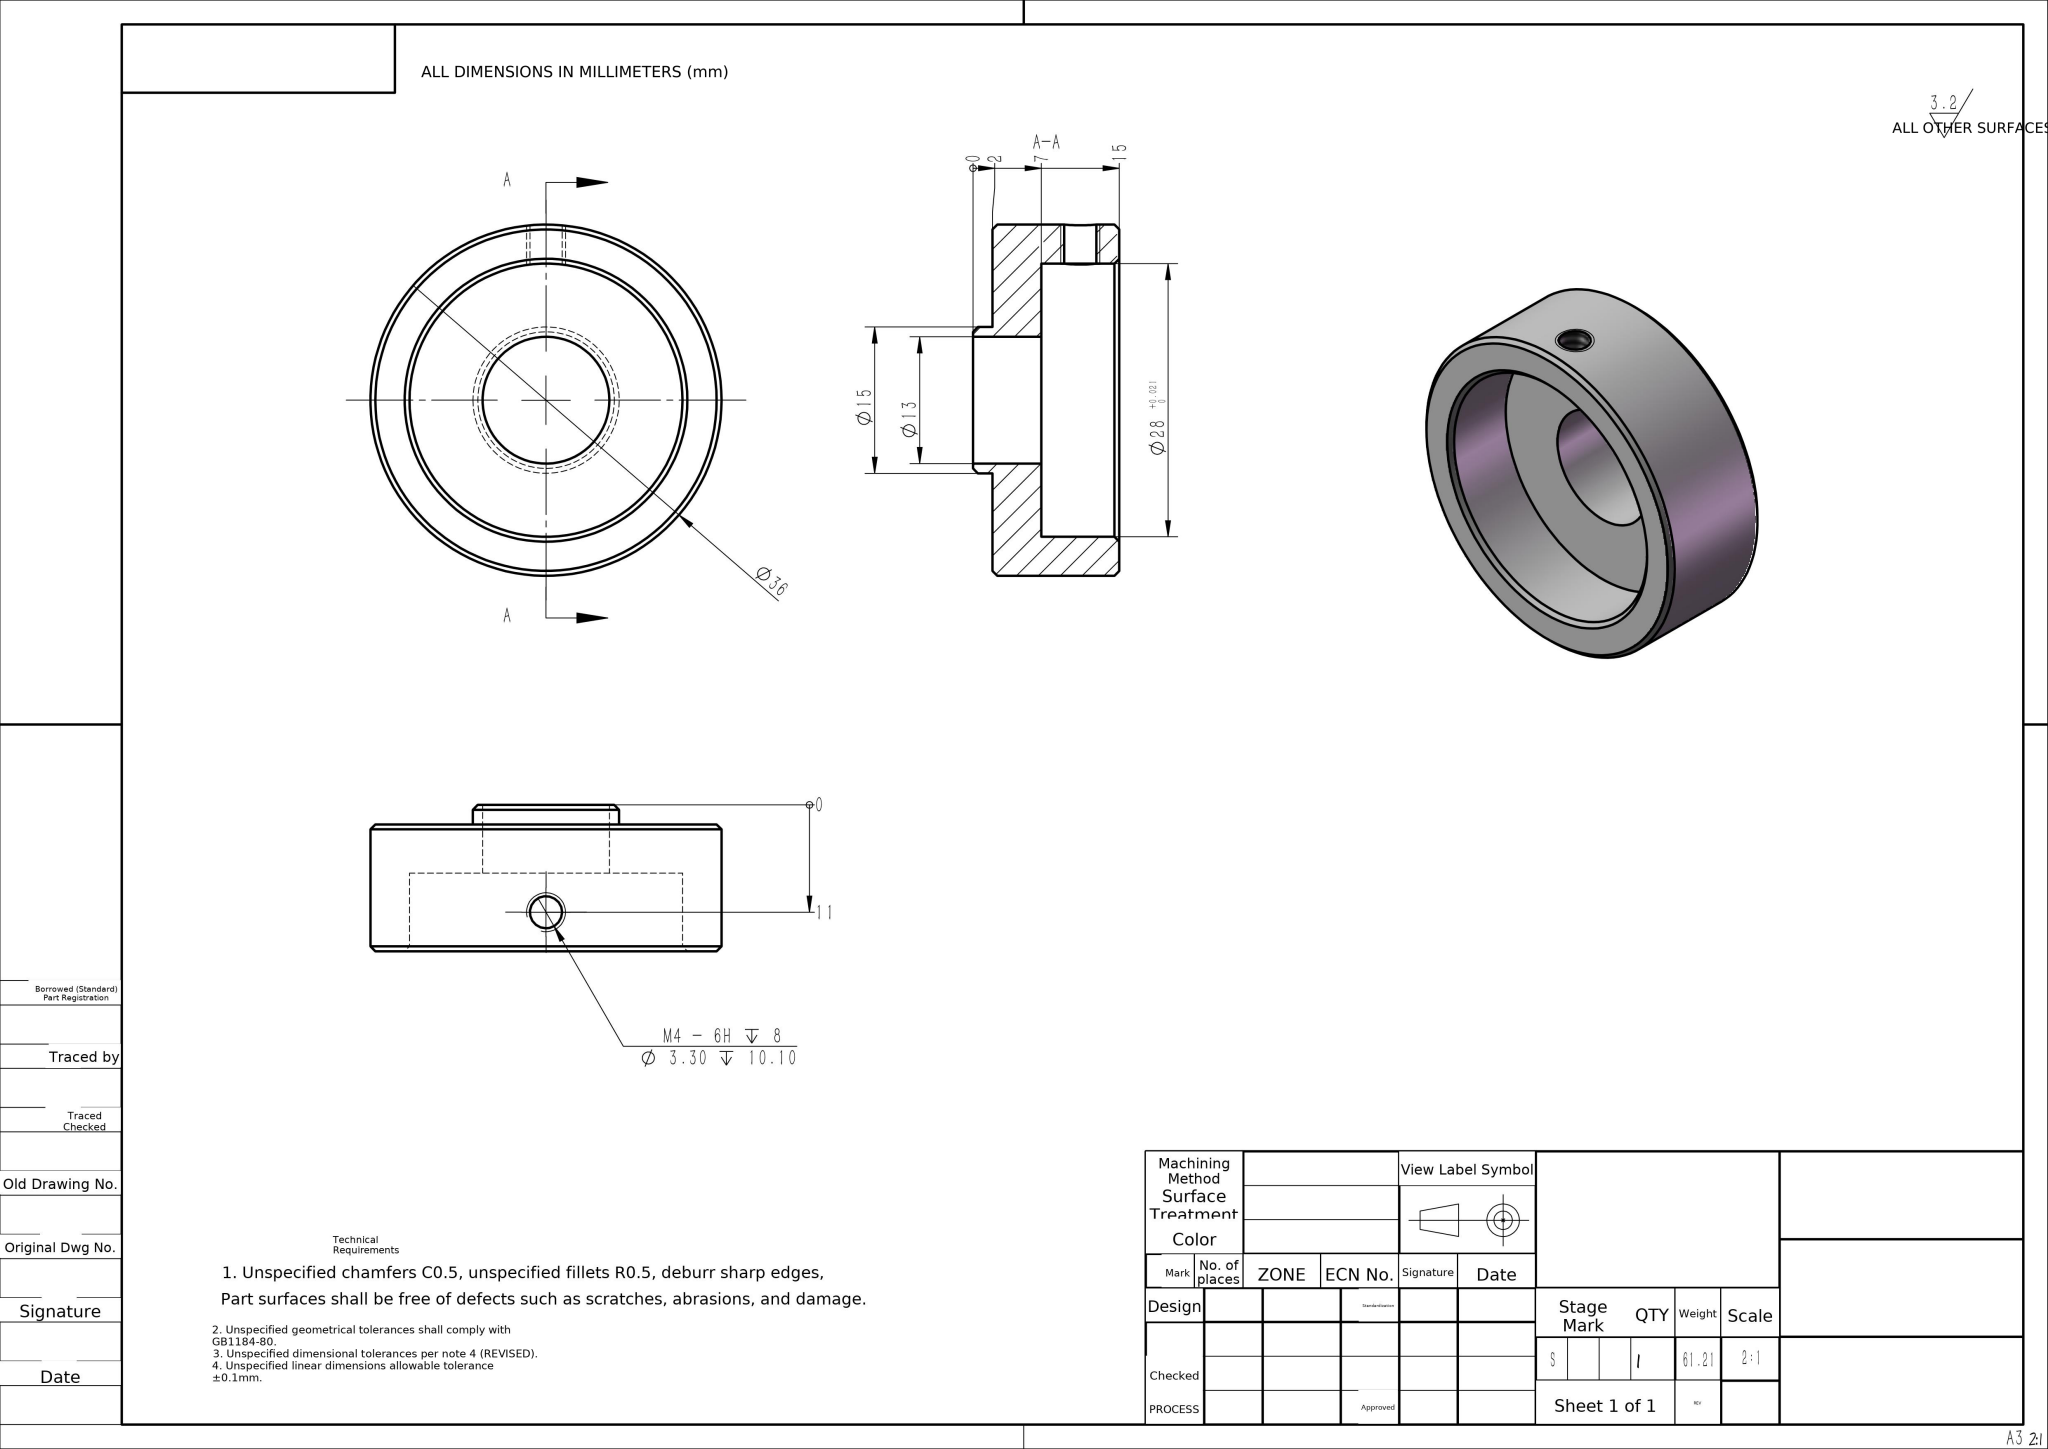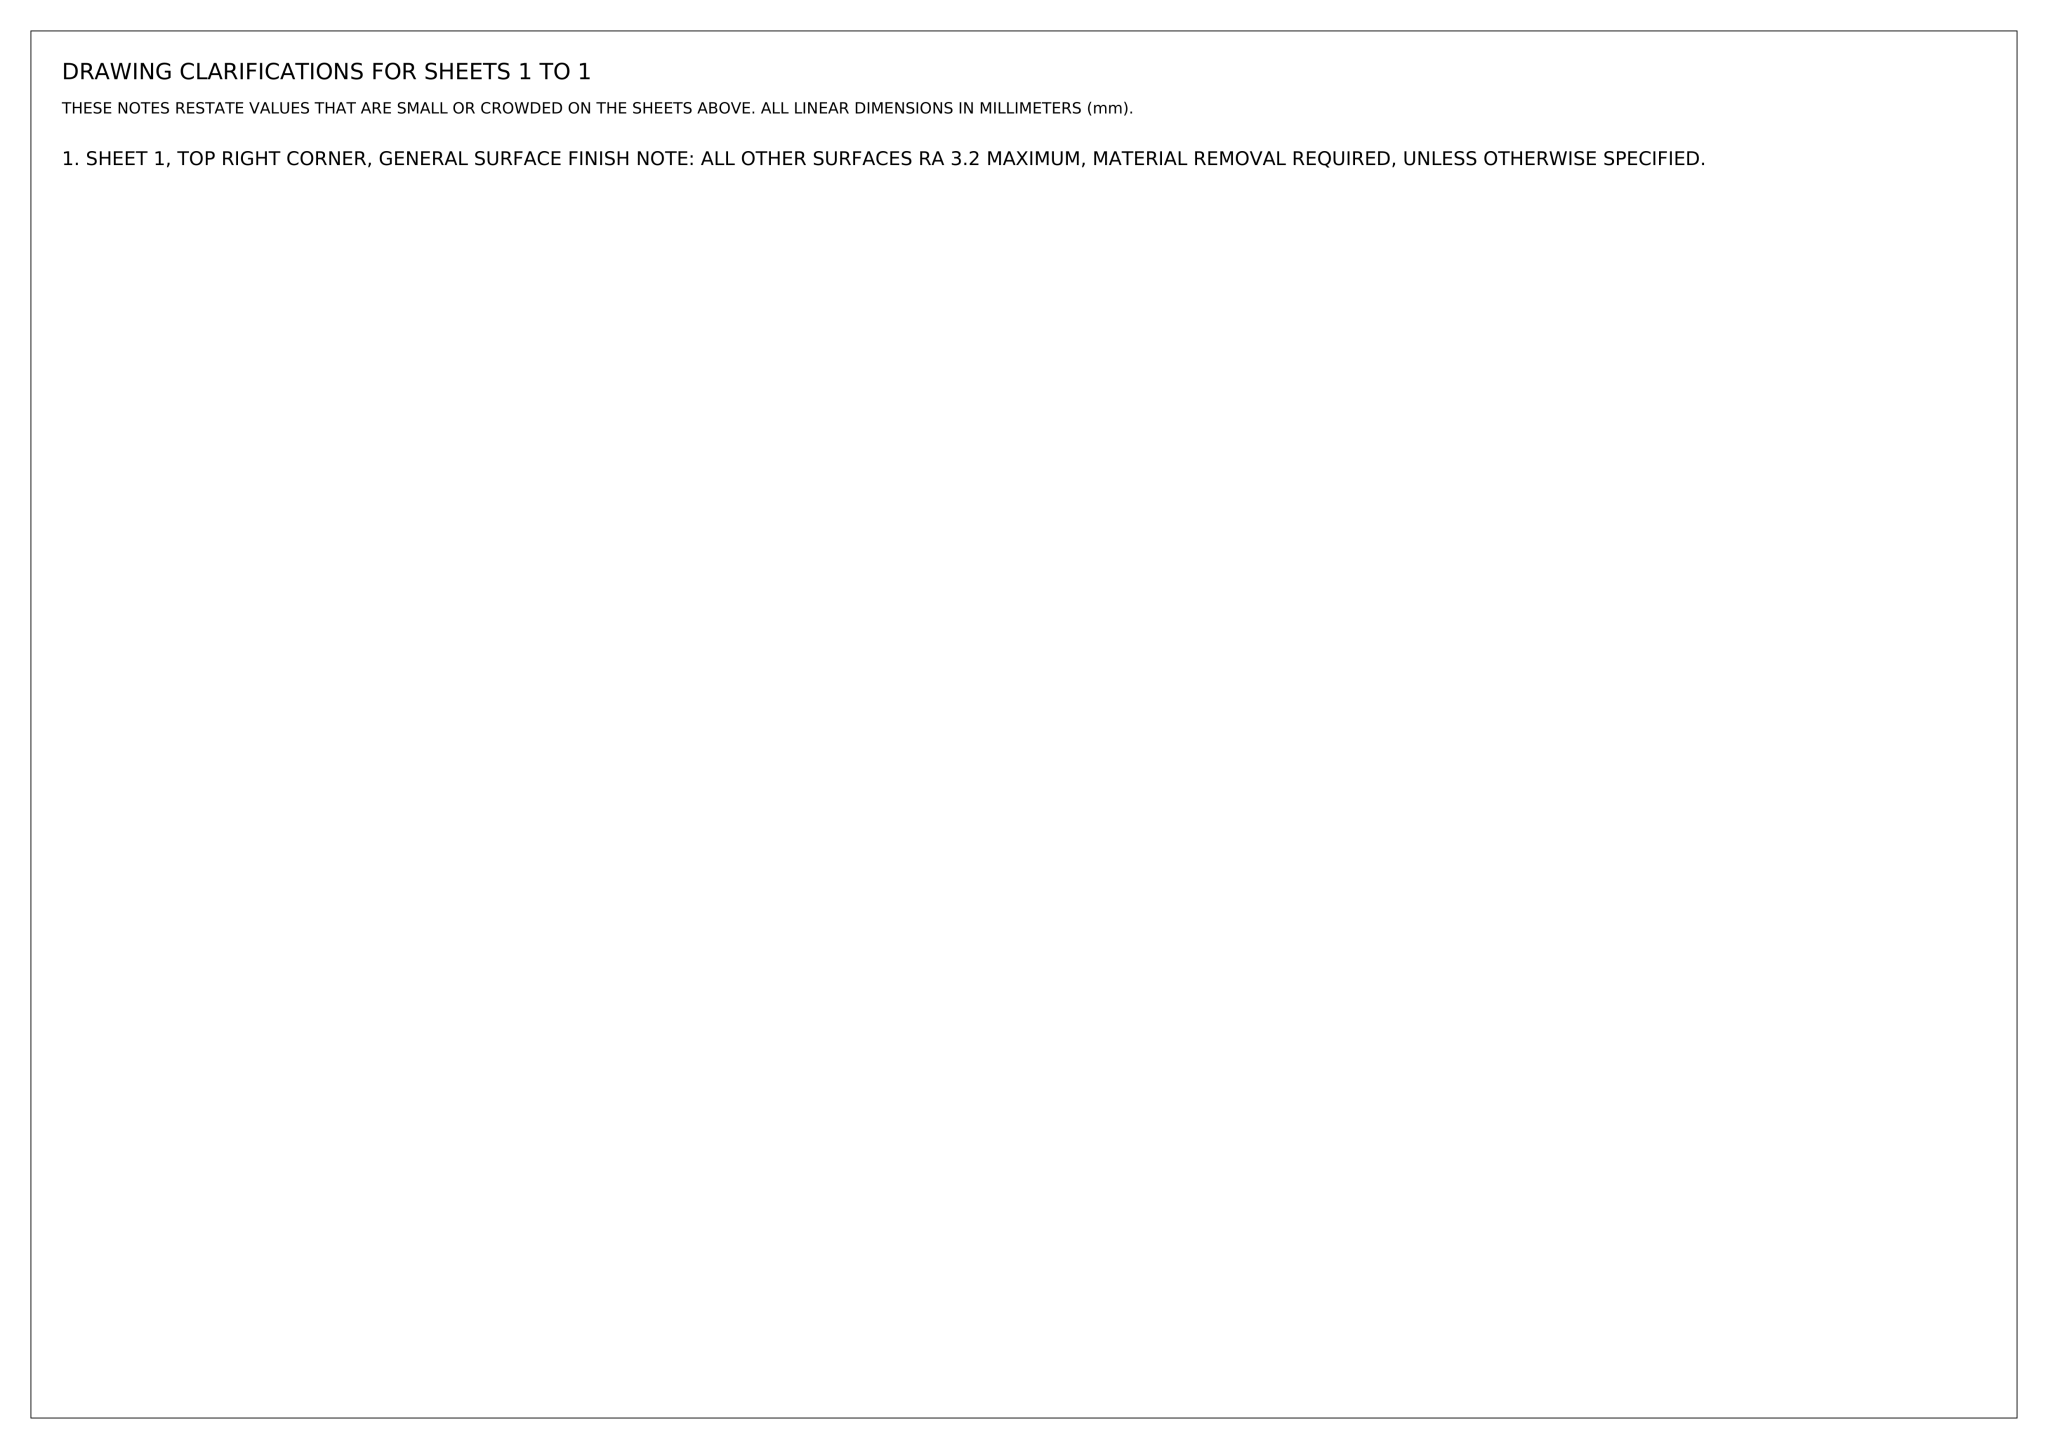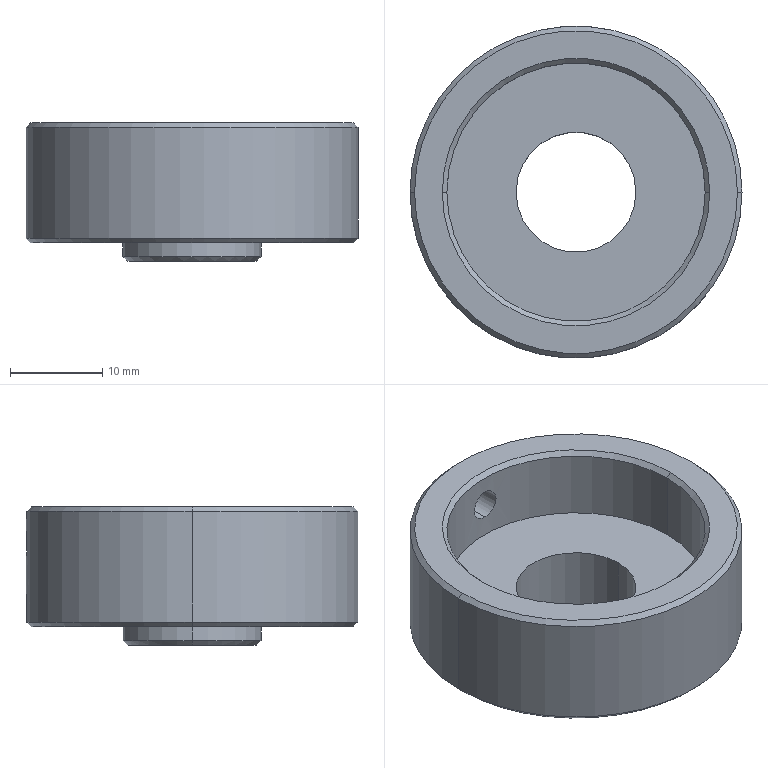Part | NX | mm | 1 solid | 22 faces | box 36 x 36 x 15 mm | volume 7652 mm3 | cylinder 10 | cone 8 | plane 4 | commonest cylinder face diameters 3.3 x2 28 x2 15 x2 36 x2 13 x2
STEP:
#1=CARTESIAN_POINT('',(0.,14.,9.35));
#2=VERTEX_POINT('',#1);
#3=CARTESIAN_POINT('',(0.,14.,12.65));
#4=VERTEX_POINT('',#3);
#5=CARTESIAN_POINT('',(0.,14.,9.35));
#6=CARTESIAN_POINT('',(-0.2154,14.,9.35));
#7=CARTESIAN_POINT('',(-0.4327,13.995,9.393));
#8=CARTESIAN_POINT('',(-0.8298,13.977,9.558));
#9=CARTESIAN_POINT('',(-1.014,13.964,9.68));
#10=CARTESIAN_POINT('',(-1.242,13.945,9.908));
#11=CARTESIAN_POINT('',(-1.312,13.939,9.993));
#12=CARTESIAN_POINT('',(-1.431,13.927,10.172));
#13=CARTESIAN_POINT('',(-1.482,13.921,10.267));
#14=CARTESIAN_POINT('',(-1.565,13.912,10.467));
#15=CARTESIAN_POINT('',(-1.597,13.909,10.572));
#16=CARTESIAN_POINT('',(-1.639,13.904,10.782));
#17=CARTESIAN_POINT('',(-1.65,13.902,10.89));
#18=CARTESIAN_POINT('',(-1.65,13.902,11.108));
#19=CARTESIAN_POINT('',(-1.639,13.904,11.215));
#20=CARTESIAN_POINT('',(-1.598,13.909,11.426));
#21=CARTESIAN_POINT('',(-1.566,13.912,11.531));
#22=CARTESIAN_POINT('',(-1.483,13.921,11.731));
#23=CARTESIAN_POINT('',(-1.433,13.927,11.826));
#24=CARTESIAN_POINT('',(-1.313,13.938,12.005));
#25=CARTESIAN_POINT('',(-1.244,13.945,12.09));
#26=CARTESIAN_POINT('',(-1.016,13.964,12.318));
#27=CARTESIAN_POINT('',(-0.8318,13.977,12.441));
#28=CARTESIAN_POINT('',(-0.435,13.995,12.606));
#29=CARTESIAN_POINT('',(-0.2182,14.,12.65));
#30=CARTESIAN_POINT('',(0.,14.,12.65));
#31=B_SPLINE_CURVE_WITH_KNOTS('',3,(#5,#6,#7,#8,#9,#10,#11,#12,#13,#14,#15,#16,#17,#18,#19,#20,#21,#22,#23,#24,#25,#26,#27,#28,#29,#30),.UNSPECIFIED.,.F.,.F.,(4,2,2,2,2,2,2,2,2,2,2,2,4),(0.005163,0.005808,0.006454,0.006776,0.007099,0.007421,0.007744,0.008067,0.008389,0.008712,0.009035,0.00968,0.01033),.UNSPECIFIED.);
#32=EDGE_CURVE('',#2,#4,#31,.T.);
#33=ORIENTED_EDGE('',*,*,#32,.F.);
#34=CARTESIAN_POINT('',(0.,18.,9.35));
#35=VERTEX_POINT('',#34);
#36=CARTESIAN_POINT('',(0.,18.,9.35));
#37=DIRECTION('',(0.,1.,0.));
#38=VECTOR('',#37,1000.);
#39=LINE('',#36,#38);
#40=EDGE_CURVE('',#2,#35,#39,.T.);
#41=ORIENTED_EDGE('',*,*,#40,.T.);
#42=CARTESIAN_POINT('',(-0.,18.,12.65));
#43=VERTEX_POINT('',#42);
#44=CARTESIAN_POINT('',(-0.,18.,12.65));
#45=CARTESIAN_POINT('',(-0.1091,18.,12.65));
#46=CARTESIAN_POINT('',(-0.2163,17.999,12.639));
#47=CARTESIAN_POINT('',(-0.4273,17.995,12.597));
#48=CARTESIAN_POINT('',(-0.5321,17.992,12.566));
#49=CARTESIAN_POINT('',(-0.7319,17.985,12.483));
#50=CARTESIAN_POINT('',(-0.8267,17.981,12.432));
#51=CARTESIAN_POINT('',(-1.006,17.972,12.312));
#52=CARTESIAN_POINT('',(-1.091,17.967,12.243));
#53=CARTESIAN_POINT('',(-1.319,17.952,12.014));
#54=CARTESIAN_POINT('',(-1.442,17.942,11.83));
#55=CARTESIAN_POINT('',(-1.607,17.928,11.433));
#56=CARTESIAN_POINT('',(-1.65,17.924,11.216));
#57=CARTESIAN_POINT('',(-1.65,17.924,10.893));
#58=CARTESIAN_POINT('',(-1.639,17.925,10.784));
#59=CARTESIAN_POINT('',(-1.597,17.929,10.572));
#60=CARTESIAN_POINT('',(-1.566,17.932,10.469));
#61=CARTESIAN_POINT('',(-1.483,17.939,10.269));
#62=CARTESIAN_POINT('',(-1.432,17.943,10.173));
#63=CARTESIAN_POINT('',(-1.312,17.952,9.994));
#64=CARTESIAN_POINT('',(-1.244,17.957,9.911));
#65=CARTESIAN_POINT('',(-1.09,17.967,9.756));
#66=CARTESIAN_POINT('',(-1.007,17.972,9.688));
#67=CARTESIAN_POINT('',(-0.8279,17.981,9.569));
#68=CARTESIAN_POINT('',(-0.7314,17.985,9.517));
#69=CARTESIAN_POINT('',(-0.5315,17.992,9.434));
#70=CARTESIAN_POINT('',(-0.4287,17.995,9.403));
#71=CARTESIAN_POINT('',(-0.2171,17.999,9.361));
#72=CARTESIAN_POINT('',(-0.1077,18.,9.35));
#73=CARTESIAN_POINT('',(0.,18.,9.35));
#74=B_SPLINE_CURVE_WITH_KNOTS('',3,(#44,#45,#46,#47,#48,#49,#50,#51,#52,#53,#54,#55,#56,#57,#58,#59,#60,#61,#62,#63,#64,#65,#66,#67,#68,#69,#70,#71,#72,#73),.UNSPECIFIED.,.F.,.F.,(4,2,2,2,2,2,2,2,2,2,2,2,2,2,4),(0.,0.0003226,0.0006452,0.0009678,0.00129,0.001936,0.002581,0.002903,0.003226,0.003548,0.003871,0.004194,0.004516,0.004839,0.005161),.UNSPECIFIED.);
#75=EDGE_CURVE('',#43,#35,#74,.T.);
#76=ORIENTED_EDGE('',*,*,#75,.F.);
#77=CARTESIAN_POINT('',(0.,18.,12.65));
#78=DIRECTION('',(0.,1.,0.));
#79=VECTOR('',#78,1000.);
#80=LINE('',#77,#79);
#81=EDGE_CURVE('',#4,#43,#80,.T.);
#82=ORIENTED_EDGE('',*,*,#81,.F.);
#83=EDGE_LOOP('',(#33,#41,#76,#82));
#84=FACE_OUTER_BOUND('',#83,.T.);
#85=CARTESIAN_POINT('',(0.,18.,11.));
#86=DIRECTION('',(0.,1.,0.));
#87=DIRECTION('',(0.,0.,1.));
#88=AXIS2_PLACEMENT_3D('',#85,#86,#87);
#89=CYLINDRICAL_SURFACE('',#88,1.65);
#90=ADVANCED_FACE('',(#84),#89,.F.);
#91=CARTESIAN_POINT('',(-7.,0.,0.));
#92=VERTEX_POINT('',#91);
#93=CARTESIAN_POINT('',(7.,0.,0.));
#94=VERTEX_POINT('',#93);
#95=CARTESIAN_POINT('',(0.,0.,0.));
#96=DIRECTION('',(0.,0.,-1.));
#97=DIRECTION('',(1.,0.,0.));
#98=AXIS2_PLACEMENT_3D('',#95,#96,#97);
#99=CIRCLE('',#98,7.);
#100=EDGE_CURVE('',#92,#94,#99,.T.);
#101=ORIENTED_EDGE('',*,*,#100,.F.);
#102=CARTESIAN_POINT('',(-7.5,0.,0.5));
#103=VERTEX_POINT('',#102);
#104=CARTESIAN_POINT('',(-7.,0.,0.));
#105=DIRECTION('',(-0.7071,0.,0.7071));
#106=VECTOR('',#105,1000.);
#107=LINE('',#104,#106);
#108=EDGE_CURVE('',#92,#103,#107,.T.);
#109=ORIENTED_EDGE('',*,*,#108,.T.);
#110=CARTESIAN_POINT('',(7.5,0.,0.5));
#111=VERTEX_POINT('',#110);
#112=CARTESIAN_POINT('',(0.,0.,0.5));
#113=DIRECTION('',(0.,0.,1.));
#114=DIRECTION('',(1.,0.,0.));
#115=AXIS2_PLACEMENT_3D('',#112,#113,#114);
#116=CIRCLE('',#115,7.5);
#117=EDGE_CURVE('',#111,#103,#116,.T.);
#118=ORIENTED_EDGE('',*,*,#117,.F.);
#119=CARTESIAN_POINT('',(7.,0.,0.));
#120=DIRECTION('',(0.7071,0.,0.7071));
#121=VECTOR('',#120,1000.);
#122=LINE('',#119,#121);
#123=EDGE_CURVE('',#94,#111,#122,.T.);
#124=ORIENTED_EDGE('',*,*,#123,.F.);
#125=EDGE_LOOP('',(#101,#109,#118,#124));
#126=FACE_OUTER_BOUND('',#125,.T.);
#127=CARTESIAN_POINT('',(0.,0.,0.));
#128=DIRECTION('',(0.,0.,1.));
#129=DIRECTION('',(1.,0.,0.));
#130=AXIS2_PLACEMENT_3D('',#127,#128,#129);
#131=CONICAL_SURFACE('',#130,7.,0.7854);
#132=ADVANCED_FACE('',(#126),#131,.T.);
#133=CARTESIAN_POINT('',(-17.5,0.,2.));
#134=VERTEX_POINT('',#133);
#135=CARTESIAN_POINT('',(17.5,0.,2.));
#136=VERTEX_POINT('',#135);
#137=CARTESIAN_POINT('',(0.,0.,2.));
#138=DIRECTION('',(0.,0.,-1.));
#139=DIRECTION('',(-1.,0.,0.));
#140=AXIS2_PLACEMENT_3D('',#137,#138,#139);
#141=CIRCLE('',#140,17.5);
#142=EDGE_CURVE('',#134,#136,#141,.T.);
#143=ORIENTED_EDGE('',*,*,#142,.F.);
#144=CARTESIAN_POINT('',(-18.,0.,2.5));
#145=VERTEX_POINT('',#144);
#146=CARTESIAN_POINT('',(-17.5,0.,2.));
#147=DIRECTION('',(-0.7071,0.,0.7071));
#148=VECTOR('',#147,1000.);
#149=LINE('',#146,#148);
#150=EDGE_CURVE('',#134,#145,#149,.T.);
#151=ORIENTED_EDGE('',*,*,#150,.T.);
#152=CARTESIAN_POINT('',(18.,0.,2.5));
#153=VERTEX_POINT('',#152);
#154=CARTESIAN_POINT('',(0.,0.,2.5));
#155=DIRECTION('',(0.,0.,1.));
#156=DIRECTION('',(-1.,0.,0.));
#157=AXIS2_PLACEMENT_3D('',#154,#155,#156);
#158=CIRCLE('',#157,18.);
#159=EDGE_CURVE('',#153,#145,#158,.T.);
#160=ORIENTED_EDGE('',*,*,#159,.F.);
#161=CARTESIAN_POINT('',(17.5,0.,2.));
#162=DIRECTION('',(0.7071,0.,0.7071));
#163=VECTOR('',#162,1000.);
#164=LINE('',#161,#163);
#165=EDGE_CURVE('',#136,#153,#164,.T.);
#166=ORIENTED_EDGE('',*,*,#165,.F.);
#167=EDGE_LOOP('',(#143,#151,#160,#166));
#168=FACE_OUTER_BOUND('',#167,.T.);
#169=CARTESIAN_POINT('',(0.,0.,2.));
#170=DIRECTION('',(0.,0.,1.));
#171=DIRECTION('',(1.,0.,0.));
#172=AXIS2_PLACEMENT_3D('',#169,#170,#171);
#173=CONICAL_SURFACE('',#172,17.5,0.7854);
#174=ADVANCED_FACE('',(#168),#173,.T.);
#175=CARTESIAN_POINT('',(17.5,0.,15.));
#176=VERTEX_POINT('',#175);
#177=CARTESIAN_POINT('',(-17.5,0.,15.));
#178=VERTEX_POINT('',#177);
#179=CARTESIAN_POINT('',(0.,0.,15.));
#180=DIRECTION('',(0.,0.,1.));
#181=DIRECTION('',(1.,0.,0.));
#182=AXIS2_PLACEMENT_3D('',#179,#180,#181);
#183=CIRCLE('',#182,17.5);
#184=EDGE_CURVE('',#176,#178,#183,.T.);
#185=ORIENTED_EDGE('',*,*,#184,.F.);
#186=CARTESIAN_POINT('',(18.,0.,14.5));
#187=VERTEX_POINT('',#186);
#188=CARTESIAN_POINT('',(17.5,0.,15.));
#189=DIRECTION('',(0.7071,0.,-0.7071));
#190=VECTOR('',#189,1000.);
#191=LINE('',#188,#190);
#192=EDGE_CURVE('',#176,#187,#191,.T.);
#193=ORIENTED_EDGE('',*,*,#192,.T.);
#194=CARTESIAN_POINT('',(-18.,0.,14.5));
#195=VERTEX_POINT('',#194);
#196=CARTESIAN_POINT('',(0.,0.,14.5));
#197=DIRECTION('',(0.,0.,-1.));
#198=DIRECTION('',(1.,0.,0.));
#199=AXIS2_PLACEMENT_3D('',#196,#197,#198);
#200=CIRCLE('',#199,18.);
#201=EDGE_CURVE('',#195,#187,#200,.T.);
#202=ORIENTED_EDGE('',*,*,#201,.F.);
#203=CARTESIAN_POINT('',(-17.5,0.,15.));
#204=DIRECTION('',(-0.7071,0.,-0.7071));
#205=VECTOR('',#204,1000.);
#206=LINE('',#203,#205);
#207=EDGE_CURVE('',#178,#195,#206,.T.);
#208=ORIENTED_EDGE('',*,*,#207,.F.);
#209=EDGE_LOOP('',(#185,#193,#202,#208));
#210=FACE_OUTER_BOUND('',#209,.T.);
#211=CARTESIAN_POINT('',(0.,0.,15.));
#212=DIRECTION('',(0.,0.,-1.));
#213=DIRECTION('',(-1.,0.,0.));
#214=AXIS2_PLACEMENT_3D('',#211,#212,#213);
#215=CONICAL_SURFACE('',#214,17.5,0.7854);
#216=ADVANCED_FACE('',(#210),#215,.T.);
#217=CARTESIAN_POINT('',(-14.,0.,14.5));
#218=VERTEX_POINT('',#217);
#219=CARTESIAN_POINT('',(14.,0.,14.5));
#220=VERTEX_POINT('',#219);
#221=CARTESIAN_POINT('',(0.,0.,14.5));
#222=DIRECTION('',(0.,0.,1.));
#223=DIRECTION('',(1.,0.,0.));
#224=AXIS2_PLACEMENT_3D('',#221,#222,#223);
#225=CIRCLE('',#224,14.);
#226=EDGE_CURVE('',#218,#220,#225,.T.);
#227=ORIENTED_EDGE('',*,*,#226,.F.);
#228=CARTESIAN_POINT('',(-14.5,0.,15.));
#229=VERTEX_POINT('',#228);
#230=CARTESIAN_POINT('',(-14.,0.,14.5));
#231=DIRECTION('',(-0.7071,0.,0.7071));
#232=VECTOR('',#231,1000.);
#233=LINE('',#230,#232);
#234=EDGE_CURVE('',#218,#229,#233,.T.);
#235=ORIENTED_EDGE('',*,*,#234,.T.);
#236=CARTESIAN_POINT('',(14.5,0.,15.));
#237=VERTEX_POINT('',#236);
#238=CARTESIAN_POINT('',(0.,0.,15.));
#239=DIRECTION('',(0.,0.,-1.));
#240=DIRECTION('',(1.,0.,0.));
#241=AXIS2_PLACEMENT_3D('',#238,#239,#240);
#242=CIRCLE('',#241,14.5);
#243=EDGE_CURVE('',#237,#229,#242,.T.);
#244=ORIENTED_EDGE('',*,*,#243,.F.);
#245=CARTESIAN_POINT('',(14.,0.,14.5));
#246=DIRECTION('',(0.7071,0.,0.7071));
#247=VECTOR('',#246,1000.);
#248=LINE('',#245,#247);
#249=EDGE_CURVE('',#220,#237,#248,.T.);
#250=ORIENTED_EDGE('',*,*,#249,.F.);
#251=EDGE_LOOP('',(#227,#235,#244,#250));
#252=FACE_OUTER_BOUND('',#251,.T.);
#253=CARTESIAN_POINT('',(0.,0.,14.5));
#254=DIRECTION('',(0.,0.,1.));
#255=DIRECTION('',(1.,0.,0.));
#256=AXIS2_PLACEMENT_3D('',#253,#254,#255);
#257=CONICAL_SURFACE('',#256,14.,0.7854);
#258=ADVANCED_FACE('',(#252),#257,.F.);
#259=CARTESIAN_POINT('',(-14.,0.,7.));
#260=VERTEX_POINT('',#259);
#261=CARTESIAN_POINT('',(14.,0.,7.));
#262=VERTEX_POINT('',#261);
#263=CARTESIAN_POINT('',(0.,0.,7.));
#264=DIRECTION('',(0.,0.,1.));
#265=DIRECTION('',(1.,0.,0.));
#266=AXIS2_PLACEMENT_3D('',#263,#264,#265);
#267=CIRCLE('',#266,14.);
#268=EDGE_CURVE('',#260,#262,#267,.T.);
#269=ORIENTED_EDGE('',*,*,#268,.F.);
#270=CARTESIAN_POINT('',(-14.,0.,7.));
#271=DIRECTION('',(0.,0.,1.));
#272=VECTOR('',#271,1000.);
#273=LINE('',#270,#272);
#274=EDGE_CURVE('',#260,#218,#273,.T.);
#275=ORIENTED_EDGE('',*,*,#274,.T.);
#276=ORIENTED_EDGE('',*,*,#226,.T.);
#277=CARTESIAN_POINT('',(14.,0.,7.));
#278=DIRECTION('',(0.,0.,1.));
#279=VECTOR('',#278,1000.);
#280=LINE('',#277,#279);
#281=EDGE_CURVE('',#262,#220,#280,.T.);
#282=ORIENTED_EDGE('',*,*,#281,.F.);
#283=EDGE_LOOP('',(#269,#275,#276,#282));
#284=FACE_OUTER_BOUND('',#283,.T.);
#285=CARTESIAN_POINT('',(0.,0.,7.));
#286=DIRECTION('',(0.,0.,1.));
#287=DIRECTION('',(1.,0.,0.));
#288=AXIS2_PLACEMENT_3D('',#285,#286,#287);
#289=CYLINDRICAL_SURFACE('',#288,14.);
#290=ADVANCED_FACE('',(#284),#289,.F.);
#291=CARTESIAN_POINT('',(-7.5,0.,2.));
#292=VERTEX_POINT('',#291);
#293=CARTESIAN_POINT('',(7.5,0.,2.));
#294=VERTEX_POINT('',#293);
#295=CARTESIAN_POINT('',(0.,0.,2.));
#296=DIRECTION('',(0.,0.,-1.));
#297=DIRECTION('',(-1.,0.,0.));
#298=AXIS2_PLACEMENT_3D('',#295,#296,#297);
#299=CIRCLE('',#298,7.5);
#300=EDGE_CURVE('',#292,#294,#299,.T.);
#301=ORIENTED_EDGE('',*,*,#300,.T.);
#302=CARTESIAN_POINT('',(7.5,0.,2.));
#303=DIRECTION('',(0.,0.,-1.));
#304=VECTOR('',#303,1000.);
#305=LINE('',#302,#304);
#306=EDGE_CURVE('',#294,#111,#305,.T.);
#307=ORIENTED_EDGE('',*,*,#306,.T.);
#308=ORIENTED_EDGE('',*,*,#117,.T.);
#309=CARTESIAN_POINT('',(-7.5,0.,2.));
#310=DIRECTION('',(0.,0.,-1.));
#311=VECTOR('',#310,1000.);
#312=LINE('',#309,#311);
#313=EDGE_CURVE('',#292,#103,#312,.T.);
#314=ORIENTED_EDGE('',*,*,#313,.F.);
#315=EDGE_LOOP('',(#301,#307,#308,#314));
#316=FACE_OUTER_BOUND('',#315,.T.);
#317=CARTESIAN_POINT('',(0.,0.,2.));
#318=DIRECTION('',(0.,0.,-1.));
#319=DIRECTION('',(-1.,0.,0.));
#320=AXIS2_PLACEMENT_3D('',#317,#318,#319);
#321=CYLINDRICAL_SURFACE('',#320,7.5);
#322=ADVANCED_FACE('',(#316),#321,.T.);
#323=ORIENTED_EDGE('',*,*,#75,.T.);
#324=CARTESIAN_POINT('',(0.,18.,9.35));
#325=CARTESIAN_POINT('',(0.2154,18.,9.35));
#326=CARTESIAN_POINT('',(0.4325,17.996,9.393));
#327=CARTESIAN_POINT('',(0.8297,17.982,9.558));
#328=CARTESIAN_POINT('',(1.014,17.972,9.68));
#329=CARTESIAN_POINT('',(1.242,17.957,9.908));
#330=CARTESIAN_POINT('',(1.312,17.952,9.993));
#331=CARTESIAN_POINT('',(1.432,17.943,10.173));
#332=CARTESIAN_POINT('',(1.482,17.939,10.267));
#333=CARTESIAN_POINT('',(1.565,17.932,10.467));
#334=CARTESIAN_POINT('',(1.597,17.929,10.572));
#335=CARTESIAN_POINT('',(1.639,17.925,10.783));
#336=CARTESIAN_POINT('',(1.65,17.924,10.89));
#337=CARTESIAN_POINT('',(1.65,17.924,11.108));
#338=CARTESIAN_POINT('',(1.639,17.925,11.215));
#339=CARTESIAN_POINT('',(1.598,17.929,11.426));
#340=CARTESIAN_POINT('',(1.566,17.932,11.531));
#341=CARTESIAN_POINT('',(1.483,17.939,11.731));
#342=CARTESIAN_POINT('',(1.433,17.943,11.826));
#343=CARTESIAN_POINT('',(1.313,17.952,12.005));
#344=CARTESIAN_POINT('',(1.244,17.957,12.09));
#345=CARTESIAN_POINT('',(1.015,17.972,12.318));
#346=CARTESIAN_POINT('',(0.8317,17.982,12.441));
#347=CARTESIAN_POINT('',(0.4348,17.996,12.606));
#348=CARTESIAN_POINT('',(0.2181,18.,12.65));
#349=CARTESIAN_POINT('',(-0.,18.,12.65));
#350=B_SPLINE_CURVE_WITH_KNOTS('',3,(#324,#325,#326,#327,#328,#329,#330,#331,#332,#333,#334,#335,#336,#337,#338,#339,#340,#341,#342,#343,#344,#345,#346,#347,#348,#349),.UNSPECIFIED.,.F.,.F.,(4,2,2,2,2,2,2,2,2,2,2,2,4),(0.005161,0.005806,0.006451,0.006774,0.007096,0.007419,0.007741,0.008064,0.008386,0.008709,0.009031,0.009676,0.01032),.UNSPECIFIED.);
#351=EDGE_CURVE('',#35,#43,#350,.T.);
#352=ORIENTED_EDGE('',*,*,#351,.T.);
#353=EDGE_LOOP('',(#323,#352));
#354=FACE_BOUND('',#353,.T.);
#355=ORIENTED_EDGE('',*,*,#201,.T.);
#356=CARTESIAN_POINT('',(18.,0.,15.));
#357=DIRECTION('',(0.,0.,-1.));
#358=VECTOR('',#357,1000.);
#359=LINE('',#356,#358);
#360=EDGE_CURVE('',#187,#153,#359,.T.);
#361=ORIENTED_EDGE('',*,*,#360,.T.);
#362=ORIENTED_EDGE('',*,*,#159,.T.);
#363=CARTESIAN_POINT('',(-18.,0.,15.));
#364=DIRECTION('',(0.,0.,-1.));
#365=VECTOR('',#364,1000.);
#366=LINE('',#363,#365);
#367=EDGE_CURVE('',#195,#145,#366,.T.);
#368=ORIENTED_EDGE('',*,*,#367,.F.);
#369=EDGE_LOOP('',(#355,#361,#362,#368));
#370=FACE_OUTER_BOUND('',#369,.T.);
#371=CARTESIAN_POINT('',(0.,0.,15.));
#372=DIRECTION('',(0.,0.,-1.));
#373=DIRECTION('',(-1.,0.,0.));
#374=AXIS2_PLACEMENT_3D('',#371,#372,#373);
#375=CYLINDRICAL_SURFACE('',#374,18.);
#376=ADVANCED_FACE('',(#354,#370),#375,.T.);
#377=CARTESIAN_POINT('',(-6.5,0.,0.));
#378=VERTEX_POINT('',#377);
#379=CARTESIAN_POINT('',(6.5,0.,0.));
#380=VERTEX_POINT('',#379);
#381=CARTESIAN_POINT('',(0.,0.,0.));
#382=DIRECTION('',(0.,0.,1.));
#383=DIRECTION('',(1.,0.,0.));
#384=AXIS2_PLACEMENT_3D('',#381,#382,#383);
#385=CIRCLE('',#384,6.5);
#386=EDGE_CURVE('',#378,#380,#385,.T.);
#387=ORIENTED_EDGE('',*,*,#386,.F.);
#388=CARTESIAN_POINT('',(-6.5,0.,7.));
#389=VERTEX_POINT('',#388);
#390=CARTESIAN_POINT('',(-6.5,0.,0.));
#391=DIRECTION('',(0.,0.,1.));
#392=VECTOR('',#391,1000.);
#393=LINE('',#390,#392);
#394=EDGE_CURVE('',#378,#389,#393,.T.);
#395=ORIENTED_EDGE('',*,*,#394,.T.);
#396=CARTESIAN_POINT('',(6.5,0.,7.));
#397=VERTEX_POINT('',#396);
#398=CARTESIAN_POINT('',(0.,0.,7.));
#399=DIRECTION('',(0.,0.,-1.));
#400=DIRECTION('',(1.,0.,0.));
#401=AXIS2_PLACEMENT_3D('',#398,#399,#400);
#402=CIRCLE('',#401,6.5);
#403=EDGE_CURVE('',#397,#389,#402,.T.);
#404=ORIENTED_EDGE('',*,*,#403,.F.);
#405=CARTESIAN_POINT('',(6.5,0.,0.));
#406=DIRECTION('',(0.,0.,1.));
#407=VECTOR('',#406,1000.);
#408=LINE('',#405,#407);
#409=EDGE_CURVE('',#380,#397,#408,.T.);
#410=ORIENTED_EDGE('',*,*,#409,.F.);
#411=EDGE_LOOP('',(#387,#395,#404,#410));
#412=FACE_OUTER_BOUND('',#411,.T.);
#413=CARTESIAN_POINT('',(0.,0.,0.));
#414=DIRECTION('',(0.,0.,1.));
#415=DIRECTION('',(1.,0.,0.));
#416=AXIS2_PLACEMENT_3D('',#413,#414,#415);
#417=CYLINDRICAL_SURFACE('',#416,6.5);
#418=ADVANCED_FACE('',(#412),#417,.F.);
#419=ORIENTED_EDGE('',*,*,#394,.F.);
#420=CARTESIAN_POINT('',(0.,0.,0.));
#421=DIRECTION('',(0.,0.,1.));
#422=DIRECTION('',(1.,0.,0.));
#423=AXIS2_PLACEMENT_3D('',#420,#421,#422);
#424=CIRCLE('',#423,6.5);
#425=EDGE_CURVE('',#380,#378,#424,.T.);
#426=ORIENTED_EDGE('',*,*,#425,.F.);
#427=ORIENTED_EDGE('',*,*,#409,.T.);
#428=CARTESIAN_POINT('',(0.,0.,7.));
#429=DIRECTION('',(0.,0.,-1.));
#430=DIRECTION('',(1.,0.,0.));
#431=AXIS2_PLACEMENT_3D('',#428,#429,#430);
#432=CIRCLE('',#431,6.5);
#433=EDGE_CURVE('',#389,#397,#432,.T.);
#434=ORIENTED_EDGE('',*,*,#433,.F.);
#435=EDGE_LOOP('',(#419,#426,#427,#434));
#436=FACE_OUTER_BOUND('',#435,.T.);
#437=CARTESIAN_POINT('',(0.,0.,0.));
#438=DIRECTION('',(0.,0.,1.));
#439=DIRECTION('',(1.,0.,0.));
#440=AXIS2_PLACEMENT_3D('',#437,#438,#439);
#441=CYLINDRICAL_SURFACE('',#440,6.5);
#442=ADVANCED_FACE('',(#436),#441,.F.);
#443=ORIENTED_EDGE('',*,*,#360,.F.);
#444=CARTESIAN_POINT('',(0.,0.,14.5));
#445=DIRECTION('',(0.,0.,-1.));
#446=DIRECTION('',(1.,0.,0.));
#447=AXIS2_PLACEMENT_3D('',#444,#445,#446);
#448=CIRCLE('',#447,18.);
#449=EDGE_CURVE('',#187,#195,#448,.T.);
#450=ORIENTED_EDGE('',*,*,#449,.T.);
#451=ORIENTED_EDGE('',*,*,#367,.T.);
#452=CARTESIAN_POINT('',(0.,0.,2.5));
#453=DIRECTION('',(0.,0.,1.));
#454=DIRECTION('',(-1.,0.,0.));
#455=AXIS2_PLACEMENT_3D('',#452,#453,#454);
#456=CIRCLE('',#455,18.);
#457=EDGE_CURVE('',#145,#153,#456,.T.);
#458=ORIENTED_EDGE('',*,*,#457,.T.);
#459=EDGE_LOOP('',(#443,#450,#451,#458));
#460=FACE_OUTER_BOUND('',#459,.T.);
#461=CARTESIAN_POINT('',(0.,0.,15.));
#462=DIRECTION('',(0.,0.,-1.));
#463=DIRECTION('',(-1.,0.,0.));
#464=AXIS2_PLACEMENT_3D('',#461,#462,#463);
#465=CYLINDRICAL_SURFACE('',#464,18.);
#466=ADVANCED_FACE('',(#460),#465,.T.);
#467=CARTESIAN_POINT('',(0.,0.,0.));
#468=DIRECTION('',(0.,0.,-1.));
#469=DIRECTION('',(1.,0.,0.));
#470=AXIS2_PLACEMENT_3D('',#467,#468,#469);
#471=CIRCLE('',#470,7.);
#472=EDGE_CURVE('',#94,#92,#471,.T.);
#473=ORIENTED_EDGE('',*,*,#472,.T.);
#474=ORIENTED_EDGE('',*,*,#100,.T.);
#475=EDGE_LOOP('',(#473,#474));
#476=FACE_OUTER_BOUND('',#475,.T.);
#477=ORIENTED_EDGE('',*,*,#425,.T.);
#478=ORIENTED_EDGE('',*,*,#386,.T.);
#479=EDGE_LOOP('',(#477,#478));
#480=FACE_BOUND('',#479,.T.);
#481=CARTESIAN_POINT('',(0.,0.,0.));
#482=DIRECTION('',(0.,0.,1.));
#483=DIRECTION('',(1.,0.,0.));
#484=AXIS2_PLACEMENT_3D('',#481,#482,#483);
#485=PLANE('',#484);
#486=ADVANCED_FACE('',(#476,#480),#485,.F.);
#487=ORIENTED_EDGE('',*,*,#243,.T.);
#488=CARTESIAN_POINT('',(0.,0.,15.));
#489=DIRECTION('',(0.,0.,-1.));
#490=DIRECTION('',(1.,0.,0.));
#491=AXIS2_PLACEMENT_3D('',#488,#489,#490);
#492=CIRCLE('',#491,14.5);
#493=EDGE_CURVE('',#229,#237,#492,.T.);
#494=ORIENTED_EDGE('',*,*,#493,.T.);
#495=EDGE_LOOP('',(#487,#494));
#496=FACE_BOUND('',#495,.T.);
#497=CARTESIAN_POINT('',(0.,0.,15.));
#498=DIRECTION('',(0.,0.,1.));
#499=DIRECTION('',(1.,0.,0.));
#500=AXIS2_PLACEMENT_3D('',#497,#498,#499);
#501=CIRCLE('',#500,17.5);
#502=EDGE_CURVE('',#178,#176,#501,.T.);
#503=ORIENTED_EDGE('',*,*,#502,.T.);
#504=ORIENTED_EDGE('',*,*,#184,.T.);
#505=EDGE_LOOP('',(#503,#504));
#506=FACE_OUTER_BOUND('',#505,.T.);
#507=CARTESIAN_POINT('',(0.,0.,15.));
#508=DIRECTION('',(0.,0.,1.));
#509=DIRECTION('',(1.,0.,0.));
#510=AXIS2_PLACEMENT_3D('',#507,#508,#509);
#511=PLANE('',#510);
#512=ADVANCED_FACE('',(#496,#506),#511,.T.);
#513=CARTESIAN_POINT('',(0.,0.,2.));
#514=DIRECTION('',(0.,0.,-1.));
#515=DIRECTION('',(-1.,0.,0.));
#516=AXIS2_PLACEMENT_3D('',#513,#514,#515);
#517=CIRCLE('',#516,17.5);
#518=EDGE_CURVE('',#136,#134,#517,.T.);
#519=ORIENTED_EDGE('',*,*,#518,.T.);
#520=ORIENTED_EDGE('',*,*,#142,.T.);
#521=EDGE_LOOP('',(#519,#520));
#522=FACE_OUTER_BOUND('',#521,.T.);
#523=ORIENTED_EDGE('',*,*,#300,.F.);
#524=CARTESIAN_POINT('',(0.,0.,2.));
#525=DIRECTION('',(0.,0.,-1.));
#526=DIRECTION('',(-1.,0.,0.));
#527=AXIS2_PLACEMENT_3D('',#524,#525,#526);
#528=CIRCLE('',#527,7.5);
#529=EDGE_CURVE('',#294,#292,#528,.T.);
#530=ORIENTED_EDGE('',*,*,#529,.F.);
#531=EDGE_LOOP('',(#523,#530));
#532=FACE_BOUND('',#531,.T.);
#533=CARTESIAN_POINT('',(0.,0.,2.));
#534=DIRECTION('',(0.,0.,-1.));
#535=DIRECTION('',(-1.,0.,0.));
#536=AXIS2_PLACEMENT_3D('',#533,#534,#535);
#537=PLANE('',#536);
#538=ADVANCED_FACE('',(#522,#532),#537,.T.);
#539=ORIENTED_EDGE('',*,*,#306,.F.);
#540=ORIENTED_EDGE('',*,*,#529,.T.);
#541=ORIENTED_EDGE('',*,*,#313,.T.);
#542=CARTESIAN_POINT('',(0.,0.,0.5));
#543=DIRECTION('',(0.,0.,1.));
#544=DIRECTION('',(1.,0.,0.));
#545=AXIS2_PLACEMENT_3D('',#542,#543,#544);
#546=CIRCLE('',#545,7.5);
#547=EDGE_CURVE('',#103,#111,#546,.T.);
#548=ORIENTED_EDGE('',*,*,#547,.T.);
#549=EDGE_LOOP('',(#539,#540,#541,#548));
#550=FACE_OUTER_BOUND('',#549,.T.);
#551=CARTESIAN_POINT('',(0.,0.,2.));
#552=DIRECTION('',(0.,0.,-1.));
#553=DIRECTION('',(-1.,0.,0.));
#554=AXIS2_PLACEMENT_3D('',#551,#552,#553);
#555=CYLINDRICAL_SURFACE('',#554,7.5);
#556=ADVANCED_FACE('',(#550),#555,.T.);
#557=CARTESIAN_POINT('',(0.,0.,7.));
#558=DIRECTION('',(0.,0.,1.));
#559=DIRECTION('',(1.,0.,0.));
#560=AXIS2_PLACEMENT_3D('',#557,#558,#559);
#561=CIRCLE('',#560,14.);
#562=EDGE_CURVE('',#262,#260,#561,.T.);
#563=ORIENTED_EDGE('',*,*,#562,.T.);
#564=ORIENTED_EDGE('',*,*,#268,.T.);
#565=EDGE_LOOP('',(#563,#564));
#566=FACE_OUTER_BOUND('',#565,.T.);
#567=ORIENTED_EDGE('',*,*,#403,.T.);
#568=ORIENTED_EDGE('',*,*,#433,.T.);
#569=EDGE_LOOP('',(#567,#568));
#570=FACE_BOUND('',#569,.T.);
#571=CARTESIAN_POINT('',(0.,0.,7.));
#572=DIRECTION('',(0.,0.,1.));
#573=DIRECTION('',(1.,0.,0.));
#574=AXIS2_PLACEMENT_3D('',#571,#572,#573);
#575=PLANE('',#574);
#576=ADVANCED_FACE('',(#566,#570),#575,.T.);
#577=ORIENTED_EDGE('',*,*,#274,.F.);
#578=ORIENTED_EDGE('',*,*,#562,.F.);
#579=ORIENTED_EDGE('',*,*,#281,.T.);
#580=CARTESIAN_POINT('',(0.,0.,14.5));
#581=DIRECTION('',(0.,0.,1.));
#582=DIRECTION('',(1.,0.,0.));
#583=AXIS2_PLACEMENT_3D('',#580,#581,#582);
#584=CIRCLE('',#583,14.);
#585=EDGE_CURVE('',#220,#218,#584,.T.);
#586=ORIENTED_EDGE('',*,*,#585,.T.);
#587=EDGE_LOOP('',(#577,#578,#579,#586));
#588=FACE_OUTER_BOUND('',#587,.T.);
#589=CARTESIAN_POINT('',(0.,14.,12.65));
#590=CARTESIAN_POINT('',(0.1091,14.,12.65));
#591=CARTESIAN_POINT('',(0.2164,13.999,12.639));
#592=CARTESIAN_POINT('',(0.4274,13.994,12.597));
#593=CARTESIAN_POINT('',(0.5323,13.99,12.566));
#594=CARTESIAN_POINT('',(0.7321,13.981,12.483));
#595=CARTESIAN_POINT('',(0.8268,13.976,12.432));
#596=CARTESIAN_POINT('',(1.006,13.964,12.312));
#597=CARTESIAN_POINT('',(1.091,13.958,12.243));
#598=CARTESIAN_POINT('',(1.319,13.939,12.014));
#599=CARTESIAN_POINT('',(1.442,13.926,11.83));
#600=CARTESIAN_POINT('',(1.607,13.908,11.433));
#601=CARTESIAN_POINT('',(1.65,13.902,11.216));
#602=CARTESIAN_POINT('',(1.65,13.902,10.893));
#603=CARTESIAN_POINT('',(1.639,13.904,10.783));
#604=CARTESIAN_POINT('',(1.597,13.909,10.572));
#605=CARTESIAN_POINT('',(1.566,13.912,10.469));
#606=CARTESIAN_POINT('',(1.483,13.921,10.269));
#607=CARTESIAN_POINT('',(1.432,13.927,10.172));
#608=CARTESIAN_POINT('',(1.312,13.939,9.994));
#609=CARTESIAN_POINT('',(1.244,13.945,9.91));
#610=CARTESIAN_POINT('',(1.09,13.958,9.756));
#611=CARTESIAN_POINT('',(1.007,13.964,9.688));
#612=CARTESIAN_POINT('',(0.828,13.976,9.569));
#613=CARTESIAN_POINT('',(0.7315,13.981,9.517));
#614=CARTESIAN_POINT('',(0.5317,13.99,9.434));
#615=CARTESIAN_POINT('',(0.4288,13.994,9.403));
#616=CARTESIAN_POINT('',(0.2172,13.999,9.361));
#617=CARTESIAN_POINT('',(0.1077,14.,9.35));
#618=CARTESIAN_POINT('',(0.,14.,9.35));
#619=B_SPLINE_CURVE_WITH_KNOTS('',3,(#589,#590,#591,#592,#593,#594,#595,#596,#597,#598,#599,#600,#601,#602,#603,#604,#605,#606,#607,#608,#609,#610,#611,#612,#613,#614,#615,#616,#617,#618),.UNSPECIFIED.,.F.,.F.,(4,2,2,2,2,2,2,2,2,2,2,2,2,2,4),(0.,0.0003227,0.0006454,0.0009681,0.001291,0.001936,0.002582,0.002904,0.003227,0.00355,0.003872,0.004195,0.004518,0.00484,0.005163),.UNSPECIFIED.);
#620=EDGE_CURVE('',#4,#2,#619,.T.);
#621=ORIENTED_EDGE('',*,*,#620,.T.);
#622=ORIENTED_EDGE('',*,*,#32,.T.);
#623=EDGE_LOOP('',(#621,#622));
#624=FACE_BOUND('',#623,.T.);
#625=CARTESIAN_POINT('',(0.,0.,7.));
#626=DIRECTION('',(0.,0.,1.));
#627=DIRECTION('',(1.,0.,0.));
#628=AXIS2_PLACEMENT_3D('',#625,#626,#627);
#629=CYLINDRICAL_SURFACE('',#628,14.);
#630=ADVANCED_FACE('',(#588,#624),#629,.F.);
#631=ORIENTED_EDGE('',*,*,#234,.F.);
#632=ORIENTED_EDGE('',*,*,#585,.F.);
#633=ORIENTED_EDGE('',*,*,#249,.T.);
#634=ORIENTED_EDGE('',*,*,#493,.F.);
#635=EDGE_LOOP('',(#631,#632,#633,#634));
#636=FACE_OUTER_BOUND('',#635,.T.);
#637=CARTESIAN_POINT('',(0.,0.,14.5));
#638=DIRECTION('',(0.,0.,1.));
#639=DIRECTION('',(1.,0.,0.));
#640=AXIS2_PLACEMENT_3D('',#637,#638,#639);
#641=CONICAL_SURFACE('',#640,14.,0.7854);
#642=ADVANCED_FACE('',(#636),#641,.F.);
#643=ORIENTED_EDGE('',*,*,#192,.F.);
#644=ORIENTED_EDGE('',*,*,#502,.F.);
#645=ORIENTED_EDGE('',*,*,#207,.T.);
#646=ORIENTED_EDGE('',*,*,#449,.F.);
#647=EDGE_LOOP('',(#643,#644,#645,#646));
#648=FACE_OUTER_BOUND('',#647,.T.);
#649=CARTESIAN_POINT('',(0.,0.,15.));
#650=DIRECTION('',(0.,0.,-1.));
#651=DIRECTION('',(-1.,0.,0.));
#652=AXIS2_PLACEMENT_3D('',#649,#650,#651);
#653=CONICAL_SURFACE('',#652,17.5,0.7854);
#654=ADVANCED_FACE('',(#648),#653,.T.);
#655=ORIENTED_EDGE('',*,*,#150,.F.);
#656=ORIENTED_EDGE('',*,*,#518,.F.);
#657=ORIENTED_EDGE('',*,*,#165,.T.);
#658=ORIENTED_EDGE('',*,*,#457,.F.);
#659=EDGE_LOOP('',(#655,#656,#657,#658));
#660=FACE_OUTER_BOUND('',#659,.T.);
#661=CARTESIAN_POINT('',(0.,0.,2.));
#662=DIRECTION('',(0.,0.,1.));
#663=DIRECTION('',(1.,0.,0.));
#664=AXIS2_PLACEMENT_3D('',#661,#662,#663);
#665=CONICAL_SURFACE('',#664,17.5,0.7854);
#666=ADVANCED_FACE('',(#660),#665,.T.);
#667=ORIENTED_EDGE('',*,*,#108,.F.);
#668=ORIENTED_EDGE('',*,*,#472,.F.);
#669=ORIENTED_EDGE('',*,*,#123,.T.);
#670=ORIENTED_EDGE('',*,*,#547,.F.);
#671=EDGE_LOOP('',(#667,#668,#669,#670));
#672=FACE_OUTER_BOUND('',#671,.T.);
#673=CARTESIAN_POINT('',(0.,0.,0.));
#674=DIRECTION('',(0.,0.,1.));
#675=DIRECTION('',(1.,0.,0.));
#676=AXIS2_PLACEMENT_3D('',#673,#674,#675);
#677=CONICAL_SURFACE('',#676,7.,0.7854);
#678=ADVANCED_FACE('',(#672),#677,.T.);
#679=ORIENTED_EDGE('',*,*,#40,.F.);
#680=ORIENTED_EDGE('',*,*,#620,.F.);
#681=ORIENTED_EDGE('',*,*,#81,.T.);
#682=ORIENTED_EDGE('',*,*,#351,.F.);
#683=EDGE_LOOP('',(#679,#680,#681,#682));
#684=FACE_OUTER_BOUND('',#683,.T.);
#685=CARTESIAN_POINT('',(0.,18.,11.));
#686=DIRECTION('',(0.,1.,0.));
#687=DIRECTION('',(0.,0.,1.));
#688=AXIS2_PLACEMENT_3D('',#685,#686,#687);
#689=CYLINDRICAL_SURFACE('',#688,1.65);
#690=ADVANCED_FACE('',(#684),#689,.F.);
#691=CLOSED_SHELL('',(#90,#132,#174,#216,#258,#290,#322,#376,#418,#442,#466,#486,#512,#538,#556,#576,#630,#642,#654,#666,#678,#690));
#692=MANIFOLD_SOLID_BREP('',#691);
#693=CARTESIAN_POINT('',(0.,0.,0.));
#694=DIRECTION('',(0.,0.,1.));
#695=DIRECTION('',(1.,0.,0.));
#696=AXIS2_PLACEMENT_3D('',#693,#694,#695);
#697=(LENGTH_UNIT()NAMED_UNIT(*)SI_UNIT(.MILLI.,.METRE.));
#698=UNCERTAINTY_MEASURE_WITH_UNIT(LENGTH_MEASURE(0.00001),#697,'','');
#699=(NAMED_UNIT(*)PLANE_ANGLE_UNIT()SI_UNIT($,.RADIAN.));
#700=(NAMED_UNIT(*)SI_UNIT($,.STERADIAN.)SOLID_ANGLE_UNIT());
#701=(GEOMETRIC_REPRESENTATION_CONTEXT(3)GLOBAL_UNCERTAINTY_ASSIGNED_CONTEXT((#698))GLOBAL_UNIT_ASSIGNED_CONTEXT((#697,#699,#700))REPRESENTATION_CONTEXT('',''));
#702=ADVANCED_BREP_SHAPE_REPRESENTATION('',(#692,#696),#701);
#703=COLOUR_RGB('',0.7922,0.8196,0.9333);
#704=FILL_AREA_STYLE_COLOUR('',#703);
#705=FILL_AREA_STYLE('',(#704));
#706=SURFACE_STYLE_FILL_AREA(#705);
#707=SURFACE_SIDE_STYLE('',(#706));
#708=SURFACE_STYLE_USAGE(.BOTH.,#707);
#709=PRESENTATION_STYLE_ASSIGNMENT((#708));
#710=STYLED_ITEM('',(#709),#692);
#711=PRESENTATION_LAYER_ASSIGNMENT('','',(#710));
#712=(LENGTH_UNIT()NAMED_UNIT(*)SI_UNIT(.MILLI.,.METRE.));
#713=UNCERTAINTY_MEASURE_WITH_UNIT(LENGTH_MEASURE(0.00001),#712,'','');
#714=(NAMED_UNIT(*)PLANE_ANGLE_UNIT()SI_UNIT($,.RADIAN.));
#715=(NAMED_UNIT(*)SI_UNIT($,.STERADIAN.)SOLID_ANGLE_UNIT());
#716=(GEOMETRIC_REPRESENTATION_CONTEXT(3)GLOBAL_UNCERTAINTY_ASSIGNED_CONTEXT((#713))GLOBAL_UNIT_ASSIGNED_CONTEXT((#712,#714,#715))REPRESENTATION_CONTEXT('',''));
#717=MECHANICAL_DESIGN_GEOMETRIC_PRESENTATION_REPRESENTATION('',(#710),#716);